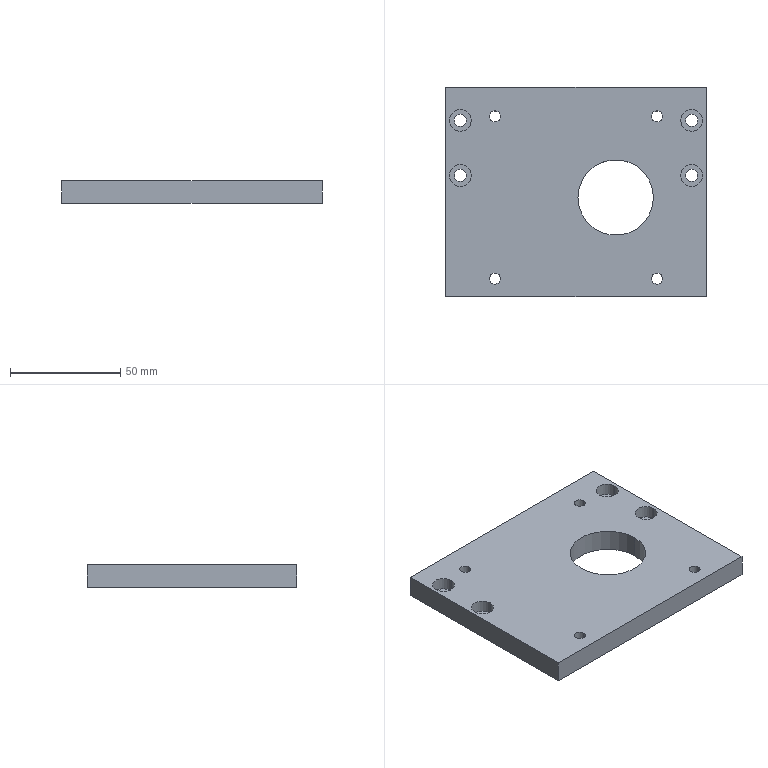Component | SolidWorks | LD101-02--Q1042-Q1-2-1 | 1 solid | 48 faces | box 118 x 95 x 10 mm | volume 99246 mm3 | cylinder 32 | plane 10 | cone 6 | commonest cylinder face diameters 5 x8 10 x8 5.5 x8 4.2 x6 34.2 x2 | material AL6061
build123d program:
from build123d import *

# Parameters (mm, degrees)
SKETCH1_W                                          = 118
SKETCH1_H                                          = 95
SKETCH1_R                                          = 17.1
BOSS_EXTRUDE1_DEPTH                                = 5
HOLE_SIZE_FOR_HEX_SOCKET_HEAD_CAP_SCRE_D           = 5.5
HOLE_SIZE_FOR_HEX_SOCKET_HEAD_CAP_SCRE_CBORE_D     = 10
HOLE_SIZE_FOR_HEX_SOCKET_HEAD_CAP_SCRE_CBORE_DEPTH = 5.7
M6_TAPPED_HOLE1_D                                  = 5
M5_TAPPED_HOLE1_D                                  = 4.2
M5_TAPPED_HOLE1_DEPTH                              = 16
M5_TAPPED_HOLE1_TIP                                = 1.262


with BuildPart() as part:
    # Sketch1 → Boss-Extrude1 (new, symmetric)
    with BuildSketch(Plane.XY):
        Rectangle(SKETCH1_W, SKETCH1_H)
        with Locations((18, -2.5)):
            Circle(SKETCH1_R, mode=Mode.SUBTRACT)
    extrude(amount=BOSS_EXTRUDE1_DEPTH, both=True)

    # Hole Size _for_ Hex Socket Head Cap Scre (through all)
    with Locations(Plane.XY.offset(5)):
        with Locations((-52.5, 7.5), (52.5, 7.5), (52.5, 32.5), (-52.5, 32.5)):
            CounterBoreHole(HOLE_SIZE_FOR_HEX_SOCKET_HEAD_CAP_SCRE_D / 2, HOLE_SIZE_FOR_HEX_SOCKET_HEAD_CAP_SCRE_CBORE_D / 2, HOLE_SIZE_FOR_HEX_SOCKET_HEAD_CAP_SCRE_CBORE_DEPTH)

    # M6 Tapped Hole1 (through all)
    with Locations(Plane.XY.offset(5)):
        with Locations((-36.77, 34.27), (-36.77, -39.27), (36.77, -39.27), (36.77, 34.27)):
            Hole(M6_TAPPED_HOLE1_D / 2)

    # M5 Tapped Hole1
    with Locations(Plane(origin=(0, 47.5, 0), x_dir=(1, 0, 0), z_dir=(0, 1, 0))):
        with Locations((0, 0), (-28, 0), (28, 0)):
            Hole(M5_TAPPED_HOLE1_D / 2, depth=M5_TAPPED_HOLE1_DEPTH)
            with Locations((0, 0, -(M5_TAPPED_HOLE1_DEPTH + M5_TAPPED_HOLE1_TIP / 2))):  # 118° drill point
                Cone(0, M5_TAPPED_HOLE1_D / 2, M5_TAPPED_HOLE1_TIP, mode=Mode.SUBTRACT)


solid = part.part

# Placed as in the assembly
solid = solid.moved(Location((229.211, -309.397, 288.257), (0, 0, 0)))